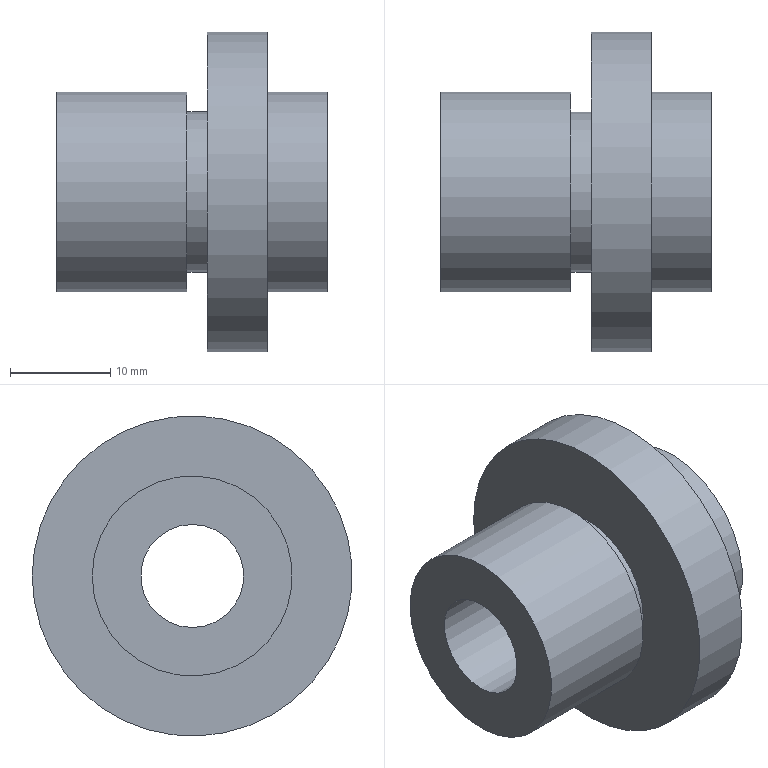Component | NX | VALVE_CAP | 1 solid | 12 faces | box 27 x 32 x 32 mm | volume 8798 mm3 | cylinder 6 | plane 6 | commonest cylinder face diameters 20 x2 32 x1 10.3 x1 16 x1 12 x1
STEP:
#1=CARTESIAN_POINT('',(0.,0.,0.));
#2=DIRECTION('',(0.,0.,1.));
#3=DIRECTION('',(1.,0.,0.));
#4=AXIS2_PLACEMENT_3D('',#1,#2,#3);
#5=CARTESIAN_POINT('',(52.,10.,20.));
#6=VERTEX_POINT('',#5);
#7=CARTESIAN_POINT('',(52.,-0.,20.));
#8=DIRECTION('',(1.,0.,0.));
#9=DIRECTION('',(0.,1.,0.));
#10=AXIS2_PLACEMENT_3D('',#7,#8,#9);
#11=CIRCLE('',#10,10.);
#12=CARTESIAN_POINT('',(67.,-0.,20.));
#13=DIRECTION('',(-1.,0.,0.));
#14=DIRECTION('',(0.,0.,1.));
#15=AXIS2_PLACEMENT_3D('',#12,#13,#14);
#16=CYLINDRICAL_SURFACE('',#15,10.);
#17=CARTESIAN_POINT('',(7.854,15.));
#18=DIRECTION('',(-1.,0.));
#19=VECTOR('',#18,1.);
#20=LINE('',#17,#19);
#21=(GEOMETRIC_REPRESENTATION_CONTEXT(2)PARAMETRIC_REPRESENTATION_CONTEXT()REPRESENTATION_CONTEXT('',''));
#22=DEFINITIONAL_REPRESENTATION('',(#20),#21);
#23=PCURVE('',#16,#22);
#24=CARTESIAN_POINT('',(52.,-0.,20.));
#25=DIRECTION('',(1.,0.,0.));
#26=DIRECTION('',(0.,0.,-1.));
#27=AXIS2_PLACEMENT_3D('',#24,#25,#26);
#28=PLANE('',#27);
#29=CARTESIAN_POINT('',(0.,0.));
#30=DIRECTION('',(0.,1.));
#31=AXIS2_PLACEMENT_2D('',#29,#30);
#32=CIRCLE('',#31,10.);
#33=(GEOMETRIC_REPRESENTATION_CONTEXT(2)PARAMETRIC_REPRESENTATION_CONTEXT()REPRESENTATION_CONTEXT('',''));
#34=DEFINITIONAL_REPRESENTATION('',(#32),#33);
#35=PCURVE('',#28,#34);
#36=SURFACE_CURVE('',#11,(#23,#35),.PCURVE_S1.);
#37=EDGE_CURVE('',#6,#6,#36,.T.);
#38=ORIENTED_EDGE('',*,*,#37,.T.);
#39=CARTESIAN_POINT('',(65.,10.,20.));
#40=VERTEX_POINT('',#39);
#41=CARTESIAN_POINT('',(65.,10.,20.));
#42=CARTESIAN_POINT('',(52.,10.,20.));
#43=B_SPLINE_CURVE_WITH_KNOTS('',1,(#41,#42),.UNSPECIFIED.,.F.,.F.,(2,2),(2.,15.),.PIECEWISE_BEZIER_KNOTS.);
#44=CARTESIAN_POINT('',(1.571,0.));
#45=DIRECTION('',(0.,1.));
#46=VECTOR('',#45,1.);
#47=LINE('',#44,#46);
#48=(GEOMETRIC_REPRESENTATION_CONTEXT(2)PARAMETRIC_REPRESENTATION_CONTEXT()REPRESENTATION_CONTEXT('',''));
#49=DEFINITIONAL_REPRESENTATION('',(#47),#48);
#50=PCURVE('',#16,#49);
#51=CARTESIAN_POINT('',(7.854,0.));
#52=DIRECTION('',(0.,1.));
#53=VECTOR('',#52,1.);
#54=LINE('',#51,#53);
#55=(GEOMETRIC_REPRESENTATION_CONTEXT(2)PARAMETRIC_REPRESENTATION_CONTEXT()REPRESENTATION_CONTEXT('',''));
#56=DEFINITIONAL_REPRESENTATION('',(#54),#55);
#57=PCURVE('',#16,#56);
#58=SEAM_CURVE('',#43,(#50,#57),.PCURVE_S1.);
#59=EDGE_CURVE('',#40,#6,#58,.T.);
#60=ORIENTED_EDGE('',*,*,#59,.F.);
#61=CARTESIAN_POINT('',(65.,-0.,20.));
#62=DIRECTION('',(1.,0.,0.));
#63=DIRECTION('',(0.,1.,0.));
#64=AXIS2_PLACEMENT_3D('',#61,#62,#63);
#65=CIRCLE('',#64,10.);
#66=CARTESIAN_POINT('',(7.854,2.));
#67=DIRECTION('',(-1.,0.));
#68=VECTOR('',#67,1.);
#69=LINE('',#66,#68);
#70=(GEOMETRIC_REPRESENTATION_CONTEXT(2)PARAMETRIC_REPRESENTATION_CONTEXT()REPRESENTATION_CONTEXT('',''));
#71=DEFINITIONAL_REPRESENTATION('',(#69),#70);
#72=PCURVE('',#16,#71);
#73=CARTESIAN_POINT('',(65.,-0.,20.));
#74=DIRECTION('',(-1.,0.,0.));
#75=DIRECTION('',(0.,0.,1.));
#76=AXIS2_PLACEMENT_3D('',#73,#74,#75);
#77=PLANE('',#76);
#78=CARTESIAN_POINT('',(0.,10.));
#79=CARTESIAN_POINT('',(17.321,10.));
#80=CARTESIAN_POINT('',(8.66,-5.));
#81=CARTESIAN_POINT('',(0.,-20.));
#82=CARTESIAN_POINT('',(-8.66,-5.));
#83=CARTESIAN_POINT('',(-17.321,10.));
#84=CARTESIAN_POINT('',(0.,10.));
#85=(BOUNDED_CURVE()B_SPLINE_CURVE(2,(#78,#79,#80,#81,#82,#83,#84),.UNSPECIFIED.,.T.,.F.)B_SPLINE_CURVE_WITH_KNOTS((1,2,2,2,2,1),(-2.094,0.,2.094,4.189,6.283,8.378),.UNSPECIFIED.)CURVE()GEOMETRIC_REPRESENTATION_ITEM()RATIONAL_B_SPLINE_CURVE((1.,0.5,1.,0.5,1.,0.5,1.))REPRESENTATION_ITEM(''));
#86=(GEOMETRIC_REPRESENTATION_CONTEXT(2)PARAMETRIC_REPRESENTATION_CONTEXT()REPRESENTATION_CONTEXT('',''));
#87=DEFINITIONAL_REPRESENTATION('',(#85),#86);
#88=PCURVE('',#77,#87);
#89=SURFACE_CURVE('',#65,(#72,#88),.PCURVE_S1.);
#90=EDGE_CURVE('',#40,#40,#89,.T.);
#91=ORIENTED_EDGE('',*,*,#90,.F.);
#92=ORIENTED_EDGE('',*,*,#59,.T.);
#93=EDGE_LOOP('',(#38,#60,#91,#92));
#94=FACE_BOUND('',#93,.T.);
#95=ADVANCED_FACE('',(#94),#16,.T.);
#96=CARTESIAN_POINT('',(52.,-0.,14.85));
#97=VERTEX_POINT('',#96);
#98=CARTESIAN_POINT('',(52.,-0.,25.15));
#99=VERTEX_POINT('',#98);
#100=CARTESIAN_POINT('',(52.,-0.,20.));
#101=DIRECTION('',(1.,0.,0.));
#102=DIRECTION('',(0.,0.,-1.));
#103=AXIS2_PLACEMENT_3D('',#100,#101,#102);
#104=CIRCLE('',#103,5.15);
#105=CARTESIAN_POINT('',(0.,0.));
#106=DIRECTION('',(1.,0.));
#107=AXIS2_PLACEMENT_2D('',#105,#106);
#108=CIRCLE('',#107,5.15);
#109=(GEOMETRIC_REPRESENTATION_CONTEXT(2)PARAMETRIC_REPRESENTATION_CONTEXT()REPRESENTATION_CONTEXT('',''));
#110=DEFINITIONAL_REPRESENTATION('',(#108),#109);
#111=PCURVE('',#28,#110);
#112=CARTESIAN_POINT('',(79.,-0.,20.));
#113=DIRECTION('',(-1.,0.,0.));
#114=DIRECTION('',(0.,0.,1.));
#115=AXIS2_PLACEMENT_3D('',#112,#113,#114);
#116=CYLINDRICAL_SURFACE('',#115,5.15);
#117=CARTESIAN_POINT('',(3.142,27.));
#118=DIRECTION('',(-1.,0.));
#119=VECTOR('',#118,1.);
#120=LINE('',#117,#119);
#121=(GEOMETRIC_REPRESENTATION_CONTEXT(2)PARAMETRIC_REPRESENTATION_CONTEXT()REPRESENTATION_CONTEXT('',''));
#122=DEFINITIONAL_REPRESENTATION('',(#120),#121);
#123=PCURVE('',#116,#122);
#124=SURFACE_CURVE('',#104,(#111,#123),.PCURVE_S1.);
#125=EDGE_CURVE('',#97,#99,#124,.T.);
#126=ORIENTED_EDGE('',*,*,#125,.T.);
#127=CARTESIAN_POINT('',(52.,-0.,20.));
#128=DIRECTION('',(1.,0.,0.));
#129=DIRECTION('',(0.,0.,-1.));
#130=AXIS2_PLACEMENT_3D('',#127,#128,#129);
#131=CIRCLE('',#130,5.15);
#132=CARTESIAN_POINT('',(0.,0.));
#133=DIRECTION('',(1.,0.));
#134=AXIS2_PLACEMENT_2D('',#132,#133);
#135=CIRCLE('',#134,5.15);
#136=(GEOMETRIC_REPRESENTATION_CONTEXT(2)PARAMETRIC_REPRESENTATION_CONTEXT()REPRESENTATION_CONTEXT('',''));
#137=DEFINITIONAL_REPRESENTATION('',(#135),#136);
#138=PCURVE('',#28,#137);
#139=CARTESIAN_POINT('',(9.425,27.));
#140=DIRECTION('',(-1.,0.));
#141=VECTOR('',#140,1.);
#142=LINE('',#139,#141);
#143=(GEOMETRIC_REPRESENTATION_CONTEXT(2)PARAMETRIC_REPRESENTATION_CONTEXT()REPRESENTATION_CONTEXT('',''));
#144=DEFINITIONAL_REPRESENTATION('',(#142),#143);
#145=PCURVE('',#116,#144);
#146=SURFACE_CURVE('',#131,(#138,#145),.PCURVE_S1.);
#147=EDGE_CURVE('',#99,#97,#146,.T.);
#148=ORIENTED_EDGE('',*,*,#147,.T.);
#149=EDGE_LOOP('',(#126,#148));
#150=FACE_BOUND('',#149,.T.);
#151=ORIENTED_EDGE('',*,*,#37,.F.);
#152=EDGE_LOOP('',(#151));
#153=FACE_BOUND('',#152,.T.);
#154=ADVANCED_FACE('',(#150,#153),#28,.F.);
#155=CARTESIAN_POINT('',(73.,16.,20.));
#156=VERTEX_POINT('',#155);
#157=CARTESIAN_POINT('',(73.,-0.,20.));
#158=DIRECTION('',(1.,0.,0.));
#159=DIRECTION('',(0.,1.,0.));
#160=AXIS2_PLACEMENT_3D('',#157,#158,#159);
#161=CIRCLE('',#160,16.);
#162=CARTESIAN_POINT('',(73.,-0.,20.));
#163=DIRECTION('',(-1.,0.,0.));
#164=DIRECTION('',(0.,0.,1.));
#165=AXIS2_PLACEMENT_3D('',#162,#163,#164);
#166=CYLINDRICAL_SURFACE('',#165,16.);
#167=CARTESIAN_POINT('',(7.854,0.));
#168=DIRECTION('',(-1.,0.));
#169=VECTOR('',#168,1.);
#170=LINE('',#167,#169);
#171=(GEOMETRIC_REPRESENTATION_CONTEXT(2)PARAMETRIC_REPRESENTATION_CONTEXT()REPRESENTATION_CONTEXT('',''));
#172=DEFINITIONAL_REPRESENTATION('',(#170),#171);
#173=PCURVE('',#166,#172);
#174=CARTESIAN_POINT('',(73.,-0.,20.));
#175=DIRECTION('',(1.,0.,0.));
#176=DIRECTION('',(0.,0.,-1.));
#177=AXIS2_PLACEMENT_3D('',#174,#175,#176);
#178=PLANE('',#177);
#179=CARTESIAN_POINT('',(0.,0.));
#180=DIRECTION('',(0.,1.));
#181=AXIS2_PLACEMENT_2D('',#179,#180);
#182=CIRCLE('',#181,16.);
#183=(GEOMETRIC_REPRESENTATION_CONTEXT(2)PARAMETRIC_REPRESENTATION_CONTEXT()REPRESENTATION_CONTEXT('',''));
#184=DEFINITIONAL_REPRESENTATION('',(#182),#183);
#185=PCURVE('',#178,#184);
#186=SURFACE_CURVE('',#161,(#173,#185),.PCURVE_S1.);
#187=EDGE_CURVE('',#156,#156,#186,.T.);
#188=ORIENTED_EDGE('',*,*,#187,.F.);
#189=CARTESIAN_POINT('',(67.,16.,20.));
#190=VERTEX_POINT('',#189);
#191=CARTESIAN_POINT('',(73.,16.,20.));
#192=CARTESIAN_POINT('',(67.,16.,20.));
#193=B_SPLINE_CURVE_WITH_KNOTS('',1,(#191,#192),.UNSPECIFIED.,.F.,.F.,(2,2),(0.,6.),.PIECEWISE_BEZIER_KNOTS.);
#194=CARTESIAN_POINT('',(7.854,0.));
#195=DIRECTION('',(0.,1.));
#196=VECTOR('',#195,1.);
#197=LINE('',#194,#196);
#198=(GEOMETRIC_REPRESENTATION_CONTEXT(2)PARAMETRIC_REPRESENTATION_CONTEXT()REPRESENTATION_CONTEXT('',''));
#199=DEFINITIONAL_REPRESENTATION('',(#197),#198);
#200=PCURVE('',#166,#199);
#201=CARTESIAN_POINT('',(1.571,0.));
#202=DIRECTION('',(0.,1.));
#203=VECTOR('',#202,1.);
#204=LINE('',#201,#203);
#205=(GEOMETRIC_REPRESENTATION_CONTEXT(2)PARAMETRIC_REPRESENTATION_CONTEXT()REPRESENTATION_CONTEXT('',''));
#206=DEFINITIONAL_REPRESENTATION('',(#204),#205);
#207=PCURVE('',#166,#206);
#208=SEAM_CURVE('',#193,(#200,#207),.PCURVE_S1.);
#209=EDGE_CURVE('',#156,#190,#208,.T.);
#210=ORIENTED_EDGE('',*,*,#209,.T.);
#211=CARTESIAN_POINT('',(67.,-0.,20.));
#212=DIRECTION('',(1.,0.,0.));
#213=DIRECTION('',(0.,1.,0.));
#214=AXIS2_PLACEMENT_3D('',#211,#212,#213);
#215=CIRCLE('',#214,16.);
#216=CARTESIAN_POINT('',(7.854,6.));
#217=DIRECTION('',(-1.,0.));
#218=VECTOR('',#217,1.);
#219=LINE('',#216,#218);
#220=(GEOMETRIC_REPRESENTATION_CONTEXT(2)PARAMETRIC_REPRESENTATION_CONTEXT()REPRESENTATION_CONTEXT('',''));
#221=DEFINITIONAL_REPRESENTATION('',(#219),#220);
#222=PCURVE('',#166,#221);
#223=CARTESIAN_POINT('',(67.,-0.,20.));
#224=DIRECTION('',(1.,0.,0.));
#225=DIRECTION('',(0.,0.,-1.));
#226=AXIS2_PLACEMENT_3D('',#223,#224,#225);
#227=PLANE('',#226);
#228=CARTESIAN_POINT('',(0.,0.));
#229=DIRECTION('',(0.,1.));
#230=AXIS2_PLACEMENT_2D('',#228,#229);
#231=CIRCLE('',#230,16.);
#232=(GEOMETRIC_REPRESENTATION_CONTEXT(2)PARAMETRIC_REPRESENTATION_CONTEXT()REPRESENTATION_CONTEXT('',''));
#233=DEFINITIONAL_REPRESENTATION('',(#231),#232);
#234=PCURVE('',#227,#233);
#235=SURFACE_CURVE('',#215,(#222,#234),.PCURVE_S1.);
#236=EDGE_CURVE('',#190,#190,#235,.T.);
#237=ORIENTED_EDGE('',*,*,#236,.T.);
#238=ORIENTED_EDGE('',*,*,#209,.F.);
#239=EDGE_LOOP('',(#188,#210,#237,#238));
#240=FACE_BOUND('',#239,.T.);
#241=ADVANCED_FACE('',(#240),#166,.T.);
#242=CARTESIAN_POINT('',(73.,10.,20.));
#243=VERTEX_POINT('',#242);
#244=CARTESIAN_POINT('',(73.,-0.,20.));
#245=DIRECTION('',(1.,0.,0.));
#246=DIRECTION('',(0.,1.,0.));
#247=AXIS2_PLACEMENT_3D('',#244,#245,#246);
#248=CIRCLE('',#247,10.);
#249=CARTESIAN_POINT('',(0.,0.));
#250=DIRECTION('',(0.,1.));
#251=AXIS2_PLACEMENT_2D('',#249,#250);
#252=CIRCLE('',#251,10.);
#253=(GEOMETRIC_REPRESENTATION_CONTEXT(2)PARAMETRIC_REPRESENTATION_CONTEXT()REPRESENTATION_CONTEXT('',''));
#254=DEFINITIONAL_REPRESENTATION('',(#252),#253);
#255=PCURVE('',#178,#254);
#256=CARTESIAN_POINT('',(79.,-0.,20.));
#257=DIRECTION('',(-1.,0.,0.));
#258=DIRECTION('',(0.,0.,1.));
#259=AXIS2_PLACEMENT_3D('',#256,#257,#258);
#260=CYLINDRICAL_SURFACE('',#259,10.);
#261=CARTESIAN_POINT('',(7.854,6.));
#262=DIRECTION('',(-1.,0.));
#263=VECTOR('',#262,1.);
#264=LINE('',#261,#263);
#265=(GEOMETRIC_REPRESENTATION_CONTEXT(2)PARAMETRIC_REPRESENTATION_CONTEXT()REPRESENTATION_CONTEXT('',''));
#266=DEFINITIONAL_REPRESENTATION('',(#264),#265);
#267=PCURVE('',#260,#266);
#268=SURFACE_CURVE('',#248,(#255,#267),.PCURVE_S1.);
#269=EDGE_CURVE('',#243,#243,#268,.T.);
#270=ORIENTED_EDGE('',*,*,#269,.F.);
#271=EDGE_LOOP('',(#270));
#272=FACE_BOUND('',#271,.T.);
#273=ORIENTED_EDGE('',*,*,#187,.T.);
#274=EDGE_LOOP('',(#273));
#275=FACE_BOUND('',#274,.T.);
#276=ADVANCED_FACE('',(#272,#275),#178,.T.);
#277=ORIENTED_EDGE('',*,*,#236,.F.);
#278=EDGE_LOOP('',(#277));
#279=FACE_BOUND('',#278,.T.);
#280=CARTESIAN_POINT('',(67.,-0.,28.));
#281=VERTEX_POINT('',#280);
#282=CARTESIAN_POINT('',(67.,-0.,20.));
#283=DIRECTION('',(1.,0.,0.));
#284=DIRECTION('',(0.,0.,1.));
#285=AXIS2_PLACEMENT_3D('',#282,#283,#284);
#286=CIRCLE('',#285,8.);
#287=CARTESIAN_POINT('',(0.,0.));
#288=DIRECTION('',(-1.,0.));
#289=AXIS2_PLACEMENT_2D('',#287,#288);
#290=CIRCLE('',#289,8.);
#291=(GEOMETRIC_REPRESENTATION_CONTEXT(2)PARAMETRIC_REPRESENTATION_CONTEXT()REPRESENTATION_CONTEXT('',''));
#292=DEFINITIONAL_REPRESENTATION('',(#290),#291);
#293=PCURVE('',#227,#292);
#294=CARTESIAN_POINT('',(67.,-0.,20.));
#295=DIRECTION('',(-1.,0.,0.));
#296=DIRECTION('',(0.,0.,1.));
#297=AXIS2_PLACEMENT_3D('',#294,#295,#296);
#298=CYLINDRICAL_SURFACE('',#297,8.);
#299=CARTESIAN_POINT('',(6.283,0.));
#300=DIRECTION('',(-1.,0.));
#301=VECTOR('',#300,1.);
#302=LINE('',#299,#301);
#303=(GEOMETRIC_REPRESENTATION_CONTEXT(2)PARAMETRIC_REPRESENTATION_CONTEXT()REPRESENTATION_CONTEXT('',''));
#304=DEFINITIONAL_REPRESENTATION('',(#302),#303);
#305=PCURVE('',#298,#304);
#306=SURFACE_CURVE('',#286,(#293,#305),.PCURVE_S1.);
#307=EDGE_CURVE('',#281,#281,#306,.T.);
#308=ORIENTED_EDGE('',*,*,#307,.T.);
#309=EDGE_LOOP('',(#308));
#310=FACE_BOUND('',#309,.T.);
#311=ADVANCED_FACE('',(#279,#310),#227,.F.);
#312=CARTESIAN_POINT('',(79.,10.,20.));
#313=VERTEX_POINT('',#312);
#314=CARTESIAN_POINT('',(79.,-0.,20.));
#315=DIRECTION('',(1.,0.,0.));
#316=DIRECTION('',(0.,1.,0.));
#317=AXIS2_PLACEMENT_3D('',#314,#315,#316);
#318=CIRCLE('',#317,10.);
#319=CARTESIAN_POINT('',(7.854,0.));
#320=DIRECTION('',(-1.,0.));
#321=VECTOR('',#320,1.);
#322=LINE('',#319,#321);
#323=(GEOMETRIC_REPRESENTATION_CONTEXT(2)PARAMETRIC_REPRESENTATION_CONTEXT()REPRESENTATION_CONTEXT('',''));
#324=DEFINITIONAL_REPRESENTATION('',(#322),#323);
#325=PCURVE('',#260,#324);
#326=CARTESIAN_POINT('',(79.,-0.,20.));
#327=DIRECTION('',(1.,0.,0.));
#328=DIRECTION('',(0.,0.,-1.));
#329=AXIS2_PLACEMENT_3D('',#326,#327,#328);
#330=PLANE('',#329);
#331=CARTESIAN_POINT('',(0.,0.));
#332=DIRECTION('',(0.,1.));
#333=AXIS2_PLACEMENT_2D('',#331,#332);
#334=CIRCLE('',#333,10.);
#335=(GEOMETRIC_REPRESENTATION_CONTEXT(2)PARAMETRIC_REPRESENTATION_CONTEXT()REPRESENTATION_CONTEXT('',''));
#336=DEFINITIONAL_REPRESENTATION('',(#334),#335);
#337=PCURVE('',#330,#336);
#338=SURFACE_CURVE('',#318,(#325,#337),.PCURVE_S1.);
#339=EDGE_CURVE('',#313,#313,#338,.T.);
#340=ORIENTED_EDGE('',*,*,#339,.F.);
#341=CARTESIAN_POINT('',(79.,10.,20.));
#342=CARTESIAN_POINT('',(73.,10.,20.));
#343=B_SPLINE_CURVE_WITH_KNOTS('',1,(#341,#342),.UNSPECIFIED.,.F.,.F.,(2,2),(0.,6.),.PIECEWISE_BEZIER_KNOTS.);
#344=CARTESIAN_POINT('',(7.854,0.));
#345=DIRECTION('',(0.,1.));
#346=VECTOR('',#345,1.);
#347=LINE('',#344,#346);
#348=(GEOMETRIC_REPRESENTATION_CONTEXT(2)PARAMETRIC_REPRESENTATION_CONTEXT()REPRESENTATION_CONTEXT('',''));
#349=DEFINITIONAL_REPRESENTATION('',(#347),#348);
#350=PCURVE('',#260,#349);
#351=CARTESIAN_POINT('',(1.571,0.));
#352=DIRECTION('',(0.,1.));
#353=VECTOR('',#352,1.);
#354=LINE('',#351,#353);
#355=(GEOMETRIC_REPRESENTATION_CONTEXT(2)PARAMETRIC_REPRESENTATION_CONTEXT()REPRESENTATION_CONTEXT('',''));
#356=DEFINITIONAL_REPRESENTATION('',(#354),#355);
#357=PCURVE('',#260,#356);
#358=SEAM_CURVE('',#343,(#350,#357),.PCURVE_S1.);
#359=EDGE_CURVE('',#313,#243,#358,.T.);
#360=ORIENTED_EDGE('',*,*,#359,.T.);
#361=ORIENTED_EDGE('',*,*,#269,.T.);
#362=ORIENTED_EDGE('',*,*,#359,.F.);
#363=EDGE_LOOP('',(#340,#360,#361,#362));
#364=FACE_BOUND('',#363,.T.);
#365=ADVANCED_FACE('',(#364),#260,.T.);
#366=CARTESIAN_POINT('',(79.,-0.,14.));
#367=VERTEX_POINT('',#366);
#368=CARTESIAN_POINT('',(79.,-0.,20.));
#369=DIRECTION('',(1.,0.,0.));
#370=DIRECTION('',(0.,0.,-1.));
#371=AXIS2_PLACEMENT_3D('',#368,#369,#370);
#372=CIRCLE('',#371,6.);
#373=CARTESIAN_POINT('',(0.,0.));
#374=DIRECTION('',(1.,0.));
#375=AXIS2_PLACEMENT_2D('',#373,#374);
#376=CIRCLE('',#375,6.);
#377=(GEOMETRIC_REPRESENTATION_CONTEXT(2)PARAMETRIC_REPRESENTATION_CONTEXT()REPRESENTATION_CONTEXT('',''));
#378=DEFINITIONAL_REPRESENTATION('',(#376),#377);
#379=PCURVE('',#330,#378);
#380=CARTESIAN_POINT('',(74.,-0.,20.));
#381=DIRECTION('',(1.,0.,0.));
#382=DIRECTION('',(0.,0.,-1.));
#383=AXIS2_PLACEMENT_3D('',#380,#381,#382);
#384=CYLINDRICAL_SURFACE('',#383,6.);
#385=CARTESIAN_POINT('',(0.,5.));
#386=DIRECTION('',(1.,0.));
#387=VECTOR('',#386,1.);
#388=LINE('',#385,#387);
#389=(GEOMETRIC_REPRESENTATION_CONTEXT(2)PARAMETRIC_REPRESENTATION_CONTEXT()REPRESENTATION_CONTEXT('',''));
#390=DEFINITIONAL_REPRESENTATION('',(#388),#389);
#391=PCURVE('',#384,#390);
#392=SURFACE_CURVE('',#372,(#379,#391),.PCURVE_S1.);
#393=EDGE_CURVE('',#367,#367,#392,.T.);
#394=ORIENTED_EDGE('',*,*,#393,.F.);
#395=EDGE_LOOP('',(#394));
#396=FACE_BOUND('',#395,.T.);
#397=ORIENTED_EDGE('',*,*,#339,.T.);
#398=EDGE_LOOP('',(#397));
#399=FACE_BOUND('',#398,.T.);
#400=ADVANCED_FACE('',(#396,#399),#330,.T.);
#401=CARTESIAN_POINT('',(74.,-0.,25.15));
#402=VERTEX_POINT('',#401);
#403=CARTESIAN_POINT('',(74.,-0.,20.));
#404=DIRECTION('',(1.,0.,0.));
#405=DIRECTION('',(0.,0.,1.));
#406=AXIS2_PLACEMENT_3D('',#403,#404,#405);
#407=CIRCLE('',#406,5.15);
#408=CARTESIAN_POINT('',(6.283,5.));
#409=DIRECTION('',(-1.,0.));
#410=VECTOR('',#409,1.);
#411=LINE('',#408,#410);
#412=(GEOMETRIC_REPRESENTATION_CONTEXT(2)PARAMETRIC_REPRESENTATION_CONTEXT()REPRESENTATION_CONTEXT('',''));
#413=DEFINITIONAL_REPRESENTATION('',(#411),#412);
#414=PCURVE('',#116,#413);
#415=CARTESIAN_POINT('',(74.,-0.,20.));
#416=DIRECTION('',(-1.,0.,0.));
#417=DIRECTION('',(0.,0.,1.));
#418=AXIS2_PLACEMENT_3D('',#415,#416,#417);
#419=PLANE('',#418);
#420=CARTESIAN_POINT('',(5.15,0.));
#421=CARTESIAN_POINT('',(5.15,-8.92));
#422=CARTESIAN_POINT('',(-2.575,-4.46));
#423=CARTESIAN_POINT('',(-10.3,-0.));
#424=CARTESIAN_POINT('',(-2.575,4.46));
#425=CARTESIAN_POINT('',(5.15,8.92));
#426=CARTESIAN_POINT('',(5.15,0.));
#427=(BOUNDED_CURVE()B_SPLINE_CURVE(2,(#420,#421,#422,#423,#424,#425,#426),.UNSPECIFIED.,.T.,.F.)B_SPLINE_CURVE_WITH_KNOTS((1,2,2,2,2,1),(-2.094,0.,2.094,4.189,6.283,8.378),.UNSPECIFIED.)CURVE()GEOMETRIC_REPRESENTATION_ITEM()RATIONAL_B_SPLINE_CURVE((1.,0.5,1.,0.5,1.,0.5,1.))REPRESENTATION_ITEM(''));
#428=(GEOMETRIC_REPRESENTATION_CONTEXT(2)PARAMETRIC_REPRESENTATION_CONTEXT()REPRESENTATION_CONTEXT('',''));
#429=DEFINITIONAL_REPRESENTATION('',(#427),#428);
#430=PCURVE('',#419,#429);
#431=SURFACE_CURVE('',#407,(#414,#430),.PCURVE_S1.);
#432=EDGE_CURVE('',#402,#402,#431,.T.);
#433=ORIENTED_EDGE('',*,*,#432,.F.);
#434=CARTESIAN_POINT('',(74.,-0.,25.15));
#435=CARTESIAN_POINT('',(52.,-0.,25.15));
#436=B_SPLINE_CURVE_WITH_KNOTS('',1,(#434,#435),.UNSPECIFIED.,.F.,.F.,(2,2),(5.,27.),.PIECEWISE_BEZIER_KNOTS.);
#437=CARTESIAN_POINT('',(6.283,0.));
#438=DIRECTION('',(0.,1.));
#439=VECTOR('',#438,1.);
#440=LINE('',#437,#439);
#441=(GEOMETRIC_REPRESENTATION_CONTEXT(2)PARAMETRIC_REPRESENTATION_CONTEXT()REPRESENTATION_CONTEXT('',''));
#442=DEFINITIONAL_REPRESENTATION('',(#440),#441);
#443=PCURVE('',#116,#442);
#444=CARTESIAN_POINT('',(0.,0.));
#445=DIRECTION('',(0.,1.));
#446=VECTOR('',#445,1.);
#447=LINE('',#444,#446);
#448=(GEOMETRIC_REPRESENTATION_CONTEXT(2)PARAMETRIC_REPRESENTATION_CONTEXT()REPRESENTATION_CONTEXT('',''));
#449=DEFINITIONAL_REPRESENTATION('',(#447),#448);
#450=PCURVE('',#116,#449);
#451=SEAM_CURVE('',#436,(#443,#450),.PCURVE_S1.);
#452=EDGE_CURVE('',#402,#99,#451,.T.);
#453=ORIENTED_EDGE('',*,*,#452,.T.);
#454=ORIENTED_EDGE('',*,*,#147,.T.);
#455=ORIENTED_EDGE('',*,*,#125,.T.);
#456=ORIENTED_EDGE('',*,*,#452,.F.);
#457=EDGE_LOOP('',(#433,#453,#454,#455,#456));
#458=FACE_BOUND('',#457,.F.);
#459=ADVANCED_FACE('',(#458),#116,.F.);
#460=CARTESIAN_POINT('',(65.,-0.,28.));
#461=VERTEX_POINT('',#460);
#462=CARTESIAN_POINT('',(65.,-0.,20.));
#463=DIRECTION('',(-1.,0.,0.));
#464=DIRECTION('',(0.,0.,1.));
#465=AXIS2_PLACEMENT_3D('',#462,#463,#464);
#466=CIRCLE('',#465,8.);
#467=CARTESIAN_POINT('',(0.,0.));
#468=DIRECTION('',(1.,0.));
#469=AXIS2_PLACEMENT_2D('',#467,#468);
#470=CIRCLE('',#469,8.);
#471=(GEOMETRIC_REPRESENTATION_CONTEXT(2)PARAMETRIC_REPRESENTATION_CONTEXT()REPRESENTATION_CONTEXT('',''));
#472=DEFINITIONAL_REPRESENTATION('',(#470),#471);
#473=PCURVE('',#77,#472);
#474=CARTESIAN_POINT('',(0.,2.));
#475=DIRECTION('',(1.,0.));
#476=VECTOR('',#475,1.);
#477=LINE('',#474,#476);
#478=(GEOMETRIC_REPRESENTATION_CONTEXT(2)PARAMETRIC_REPRESENTATION_CONTEXT()REPRESENTATION_CONTEXT('',''));
#479=DEFINITIONAL_REPRESENTATION('',(#477),#478);
#480=PCURVE('',#298,#479);
#481=SURFACE_CURVE('',#466,(#473,#480),.PCURVE_S1.);
#482=EDGE_CURVE('',#461,#461,#481,.T.);
#483=ORIENTED_EDGE('',*,*,#482,.T.);
#484=EDGE_LOOP('',(#483));
#485=FACE_BOUND('',#484,.T.);
#486=ORIENTED_EDGE('',*,*,#90,.T.);
#487=EDGE_LOOP('',(#486));
#488=FACE_BOUND('',#487,.T.);
#489=ADVANCED_FACE('',(#485,#488),#77,.F.);
#490=ORIENTED_EDGE('',*,*,#307,.F.);
#491=CARTESIAN_POINT('',(67.,-0.,28.));
#492=CARTESIAN_POINT('',(65.,-0.,28.));
#493=B_SPLINE_CURVE_WITH_KNOTS('',1,(#491,#492),.UNSPECIFIED.,.F.,.F.,(2,2),(0.,2.),.PIECEWISE_BEZIER_KNOTS.);
#494=CARTESIAN_POINT('',(6.283,0.));
#495=DIRECTION('',(0.,1.));
#496=VECTOR('',#495,1.);
#497=LINE('',#494,#496);
#498=(GEOMETRIC_REPRESENTATION_CONTEXT(2)PARAMETRIC_REPRESENTATION_CONTEXT()REPRESENTATION_CONTEXT('',''));
#499=DEFINITIONAL_REPRESENTATION('',(#497),#498);
#500=PCURVE('',#298,#499);
#501=CARTESIAN_POINT('',(0.,0.));
#502=DIRECTION('',(0.,1.));
#503=VECTOR('',#502,1.);
#504=LINE('',#501,#503);
#505=(GEOMETRIC_REPRESENTATION_CONTEXT(2)PARAMETRIC_REPRESENTATION_CONTEXT()REPRESENTATION_CONTEXT('',''));
#506=DEFINITIONAL_REPRESENTATION('',(#504),#505);
#507=PCURVE('',#298,#506);
#508=SEAM_CURVE('',#493,(#500,#507),.PCURVE_S1.);
#509=EDGE_CURVE('',#281,#461,#508,.T.);
#510=ORIENTED_EDGE('',*,*,#509,.T.);
#511=ORIENTED_EDGE('',*,*,#482,.F.);
#512=ORIENTED_EDGE('',*,*,#509,.F.);
#513=EDGE_LOOP('',(#490,#510,#511,#512));
#514=FACE_BOUND('',#513,.T.);
#515=ADVANCED_FACE('',(#514),#298,.T.);
#516=CARTESIAN_POINT('',(74.,-0.,14.));
#517=VERTEX_POINT('',#516);
#518=CARTESIAN_POINT('',(74.,-0.,20.));
#519=DIRECTION('',(-1.,0.,0.));
#520=DIRECTION('',(0.,0.,-1.));
#521=AXIS2_PLACEMENT_3D('',#518,#519,#520);
#522=CIRCLE('',#521,6.);
#523=CARTESIAN_POINT('',(0.,0.));
#524=DIRECTION('',(-1.,0.));
#525=AXIS2_PLACEMENT_2D('',#523,#524);
#526=CIRCLE('',#525,6.);
#527=(GEOMETRIC_REPRESENTATION_CONTEXT(2)PARAMETRIC_REPRESENTATION_CONTEXT()REPRESENTATION_CONTEXT('',''));
#528=DEFINITIONAL_REPRESENTATION('',(#526),#527);
#529=PCURVE('',#419,#528);
#530=CARTESIAN_POINT('',(6.283,0.));
#531=DIRECTION('',(-1.,0.));
#532=VECTOR('',#531,1.);
#533=LINE('',#530,#532);
#534=(GEOMETRIC_REPRESENTATION_CONTEXT(2)PARAMETRIC_REPRESENTATION_CONTEXT()REPRESENTATION_CONTEXT('',''));
#535=DEFINITIONAL_REPRESENTATION('',(#533),#534);
#536=PCURVE('',#384,#535);
#537=SURFACE_CURVE('',#522,(#529,#536),.PCURVE_S1.);
#538=EDGE_CURVE('',#517,#517,#537,.T.);
#539=ORIENTED_EDGE('',*,*,#538,.F.);
#540=EDGE_LOOP('',(#539));
#541=FACE_BOUND('',#540,.T.);
#542=ORIENTED_EDGE('',*,*,#432,.F.);
#543=EDGE_LOOP('',(#542));
#544=FACE_BOUND('',#543,.T.);
#545=ADVANCED_FACE('',(#541,#544),#419,.F.);
#546=ORIENTED_EDGE('',*,*,#393,.F.);
#547=CARTESIAN_POINT('',(74.,-0.,14.));
#548=CARTESIAN_POINT('',(79.,-0.,14.));
#549=B_SPLINE_CURVE_WITH_KNOTS('',1,(#547,#548),.UNSPECIFIED.,.F.,.F.,(2,2),(0.,5.),.PIECEWISE_BEZIER_KNOTS.);
#550=CARTESIAN_POINT('',(0.,0.));
#551=DIRECTION('',(0.,1.));
#552=VECTOR('',#551,1.);
#553=LINE('',#550,#552);
#554=(GEOMETRIC_REPRESENTATION_CONTEXT(2)PARAMETRIC_REPRESENTATION_CONTEXT()REPRESENTATION_CONTEXT('',''));
#555=DEFINITIONAL_REPRESENTATION('',(#553),#554);
#556=PCURVE('',#384,#555);
#557=CARTESIAN_POINT('',(6.283,0.));
#558=DIRECTION('',(0.,1.));
#559=VECTOR('',#558,1.);
#560=LINE('',#557,#559);
#561=(GEOMETRIC_REPRESENTATION_CONTEXT(2)PARAMETRIC_REPRESENTATION_CONTEXT()REPRESENTATION_CONTEXT('',''));
#562=DEFINITIONAL_REPRESENTATION('',(#560),#561);
#563=PCURVE('',#384,#562);
#564=SEAM_CURVE('',#549,(#556,#563),.PCURVE_S1.);
#565=EDGE_CURVE('',#517,#367,#564,.T.);
#566=ORIENTED_EDGE('',*,*,#565,.F.);
#567=ORIENTED_EDGE('',*,*,#538,.F.);
#568=ORIENTED_EDGE('',*,*,#565,.T.);
#569=EDGE_LOOP('',(#546,#566,#567,#568));
#570=FACE_BOUND('',#569,.F.);
#571=ADVANCED_FACE('',(#570),#384,.F.);
#572=CLOSED_SHELL('',(#95,#154,#241,#276,#311,#365,#400,#459,#489,#515,#545,#571));
#573=MANIFOLD_SOLID_BREP('',#572);
#574=(LENGTH_UNIT()NAMED_UNIT(*)SI_UNIT(.MILLI.,.METRE.));
#575=UNCERTAINTY_MEASURE_WITH_UNIT(LENGTH_MEASURE(0.00001),#574,'','');
#576=(NAMED_UNIT(*)PLANE_ANGLE_UNIT()SI_UNIT($,.RADIAN.));
#577=(NAMED_UNIT(*)SI_UNIT($,.STERADIAN.)SOLID_ANGLE_UNIT());
#578=(GEOMETRIC_REPRESENTATION_CONTEXT(3)GLOBAL_UNCERTAINTY_ASSIGNED_CONTEXT((#575))GLOBAL_UNIT_ASSIGNED_CONTEXT((#574,#576,#577))REPRESENTATION_CONTEXT('',''));
#579=ADVANCED_BREP_SHAPE_REPRESENTATION('',(#4,#573),#578);